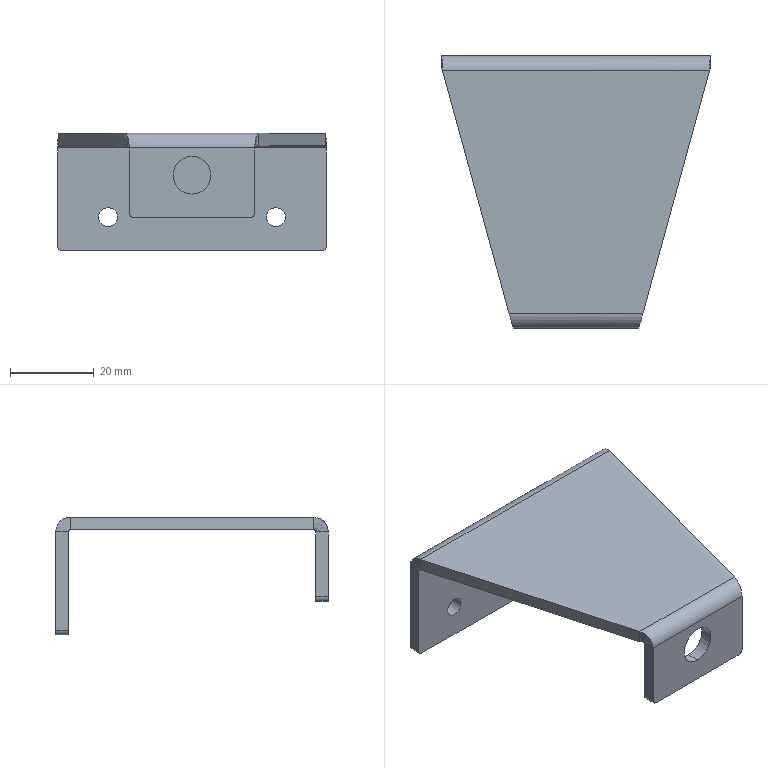Component | SolidWorks | SmallRoundCylinderBracket-1 | 1 solid | 32 faces | box 64 x 65 x 28 mm | volume 15113 mm3 | cylinder 14 | plane 14 | spline 4 | commonest cylinder face diameters 4.5 x4 2 x4 9 x2 7 x2 1 x2
STEP:
#1=CARTESIAN_POINT('',(2.534,-4.57,6.749));
#2=VERTEX_POINT('',#1);
#3=CARTESIAN_POINT('',(2.534,-4.57,6.395));
#4=VERTEX_POINT('',#3);
#5=CARTESIAN_POINT('',(2.534,-4.57,6.572));
#6=DIRECTION('',(0.,-1.,-0.));
#7=DIRECTION('',(0.,0.,-1.));
#8=AXIS2_PLACEMENT_3D('',#5,#6,#7);
#9=CIRCLE('',#8,0.1772);
#10=EDGE_CURVE('',#2,#4,#9,.T.);
#11=ORIENTED_EDGE('',*,*,#10,.F.);
#12=CARTESIAN_POINT('',(2.534,-4.688,6.749));
#13=VERTEX_POINT('',#12);
#14=CARTESIAN_POINT('',(2.534,-4.294,6.749));
#15=DIRECTION('',(0.,-1.,-0.));
#16=VECTOR('',#15,39.37);
#17=LINE('',#14,#16);
#18=EDGE_CURVE('',#2,#13,#17,.T.);
#19=ORIENTED_EDGE('',*,*,#18,.T.);
#20=CARTESIAN_POINT('',(2.534,-4.688,6.395));
#21=VERTEX_POINT('',#20);
#22=CARTESIAN_POINT('',(2.534,-4.688,6.572));
#23=DIRECTION('',(0.,-1.,-0.));
#24=DIRECTION('',(0.,0.,-1.));
#25=AXIS2_PLACEMENT_3D('',#22,#23,#24);
#26=CIRCLE('',#25,0.1772);
#27=EDGE_CURVE('',#13,#21,#26,.T.);
#28=ORIENTED_EDGE('',*,*,#27,.T.);
#29=CARTESIAN_POINT('',(2.534,-4.294,6.395));
#30=DIRECTION('',(0.,-1.,-0.));
#31=VECTOR('',#30,39.37);
#32=LINE('',#29,#31);
#33=EDGE_CURVE('',#4,#21,#32,.T.);
#34=ORIENTED_EDGE('',*,*,#33,.F.);
#35=EDGE_LOOP('',(#11,#19,#28,#34));
#36=FACE_OUTER_BOUND('',#35,.T.);
#37=CARTESIAN_POINT('',(2.534,-4.294,6.572));
#38=DIRECTION('',(0.,-1.,-0.));
#39=DIRECTION('',(0.,0.,-1.));
#40=AXIS2_PLACEMENT_3D('',#37,#38,#39);
#41=CYLINDRICAL_SURFACE('',#40,0.1772);
#42=ADVANCED_FACE('',(#36),#41,.F.);
#43=CARTESIAN_POINT('',(1.658,-2.247,6.178));
#44=VERTEX_POINT('',#43);
#45=CARTESIAN_POINT('',(1.835,-2.247,6.178));
#46=VERTEX_POINT('',#45);
#47=CARTESIAN_POINT('',(1.746,-2.247,6.178));
#48=DIRECTION('',(0.,1.,0.));
#49=DIRECTION('',(1.,0.,0.));
#50=AXIS2_PLACEMENT_3D('',#47,#48,#49);
#51=CIRCLE('',#50,0.08858);
#52=EDGE_CURVE('',#44,#46,#51,.T.);
#53=ORIENTED_EDGE('',*,*,#52,.F.);
#54=CARTESIAN_POINT('',(1.658,-2.129,6.178));
#55=VERTEX_POINT('',#54);
#56=CARTESIAN_POINT('',(1.658,-2.522,6.178));
#57=DIRECTION('',(0.,1.,0.));
#58=VECTOR('',#57,39.37);
#59=LINE('',#56,#58);
#60=EDGE_CURVE('',#44,#55,#59,.T.);
#61=ORIENTED_EDGE('',*,*,#60,.T.);
#62=CARTESIAN_POINT('',(1.835,-2.129,6.178));
#63=VERTEX_POINT('',#62);
#64=CARTESIAN_POINT('',(1.746,-2.129,6.178));
#65=DIRECTION('',(0.,1.,0.));
#66=DIRECTION('',(1.,0.,0.));
#67=AXIS2_PLACEMENT_3D('',#64,#65,#66);
#68=CIRCLE('',#67,0.08858);
#69=EDGE_CURVE('',#55,#63,#68,.T.);
#70=ORIENTED_EDGE('',*,*,#69,.T.);
#71=CARTESIAN_POINT('',(1.835,-2.522,6.178));
#72=DIRECTION('',(0.,1.,0.));
#73=VECTOR('',#72,39.37);
#74=LINE('',#71,#73);
#75=EDGE_CURVE('',#46,#63,#74,.T.);
#76=ORIENTED_EDGE('',*,*,#75,.F.);
#77=EDGE_LOOP('',(#53,#61,#70,#76));
#78=FACE_OUTER_BOUND('',#77,.T.);
#79=CARTESIAN_POINT('',(1.746,-2.522,6.178));
#80=DIRECTION('',(0.,1.,0.));
#81=DIRECTION('',(1.,0.,0.));
#82=AXIS2_PLACEMENT_3D('',#79,#80,#81);
#83=CYLINDRICAL_SURFACE('',#82,0.08858);
#84=ADVANCED_FACE('',(#78),#83,.F.);
#85=CARTESIAN_POINT('',(3.232,-2.247,6.178));
#86=VERTEX_POINT('',#85);
#87=CARTESIAN_POINT('',(3.41,-2.247,6.178));
#88=VERTEX_POINT('',#87);
#89=CARTESIAN_POINT('',(3.321,-2.247,6.178));
#90=DIRECTION('',(0.,1.,0.));
#91=DIRECTION('',(1.,0.,0.));
#92=AXIS2_PLACEMENT_3D('',#89,#90,#91);
#93=CIRCLE('',#92,0.08858);
#94=EDGE_CURVE('',#86,#88,#93,.T.);
#95=ORIENTED_EDGE('',*,*,#94,.F.);
#96=CARTESIAN_POINT('',(3.232,-2.129,6.178));
#97=VERTEX_POINT('',#96);
#98=CARTESIAN_POINT('',(3.232,-2.522,6.178));
#99=DIRECTION('',(0.,1.,0.));
#100=VECTOR('',#99,39.37);
#101=LINE('',#98,#100);
#102=EDGE_CURVE('',#86,#97,#101,.T.);
#103=ORIENTED_EDGE('',*,*,#102,.T.);
#104=CARTESIAN_POINT('',(3.41,-2.129,6.178));
#105=VERTEX_POINT('',#104);
#106=CARTESIAN_POINT('',(3.321,-2.129,6.178));
#107=DIRECTION('',(0.,1.,0.));
#108=DIRECTION('',(1.,0.,0.));
#109=AXIS2_PLACEMENT_3D('',#106,#107,#108);
#110=CIRCLE('',#109,0.08858);
#111=EDGE_CURVE('',#97,#105,#110,.T.);
#112=ORIENTED_EDGE('',*,*,#111,.T.);
#113=CARTESIAN_POINT('',(3.41,-2.522,6.178));
#114=DIRECTION('',(0.,1.,0.));
#115=VECTOR('',#114,39.37);
#116=LINE('',#113,#115);
#117=EDGE_CURVE('',#88,#105,#116,.T.);
#118=ORIENTED_EDGE('',*,*,#117,.F.);
#119=EDGE_LOOP('',(#95,#103,#112,#118));
#120=FACE_OUTER_BOUND('',#119,.T.);
#121=CARTESIAN_POINT('',(3.321,-2.522,6.178));
#122=DIRECTION('',(0.,1.,0.));
#123=DIRECTION('',(1.,0.,0.));
#124=AXIS2_PLACEMENT_3D('',#121,#122,#123);
#125=CYLINDRICAL_SURFACE('',#124,0.08858);
#126=ADVANCED_FACE('',(#120),#125,.F.);
#127=CARTESIAN_POINT('',(3.793,-2.129,6.828));
#128=VERTEX_POINT('',#127);
#129=CARTESIAN_POINT('',(1.274,-2.129,6.828));
#130=VERTEX_POINT('',#129);
#131=CARTESIAN_POINT('',(3.793,-2.129,6.828));
#132=DIRECTION('',(-1.,0.,0.));
#133=VECTOR('',#132,39.37);
#134=LINE('',#131,#133);
#135=EDGE_CURVE('',#128,#130,#134,.T.);
#136=ORIENTED_EDGE('',*,*,#135,.T.);
#137=CARTESIAN_POINT('',(1.279,-2.266,6.966));
#138=VERTEX_POINT('',#137);
#139=CARTESIAN_POINT('',(1.279,-2.266,6.966));
#140=CARTESIAN_POINT('',(1.276,-2.186,6.966));
#141=CARTESIAN_POINT('',(1.274,-2.129,6.909));
#142=CARTESIAN_POINT('',(1.274,-2.129,6.828));
#143=(BOUNDED_CURVE()B_SPLINE_CURVE(3,(#139,#140,#141,#142),.UNSPECIFIED.,.F.,.F.)B_SPLINE_CURVE_WITH_KNOTS((4,4),(4.712,6.283),.UNSPECIFIED.)CURVE()GEOMETRIC_REPRESENTATION_ITEM()RATIONAL_B_SPLINE_CURVE((1.,0.8047,0.8047,1.))REPRESENTATION_ITEM(''));
#144=EDGE_CURVE('',#138,#130,#143,.T.);
#145=ORIENTED_EDGE('',*,*,#144,.F.);
#146=CARTESIAN_POINT('',(3.788,-2.266,6.966));
#147=VERTEX_POINT('',#146);
#148=CARTESIAN_POINT('',(3.793,-2.266,6.966));
#149=DIRECTION('',(-1.,0.,0.));
#150=VECTOR('',#149,39.37);
#151=LINE('',#148,#150);
#152=EDGE_CURVE('',#147,#138,#151,.T.);
#153=ORIENTED_EDGE('',*,*,#152,.F.);
#154=CARTESIAN_POINT('',(3.793,-2.129,6.828));
#155=CARTESIAN_POINT('',(3.793,-2.129,6.909));
#156=CARTESIAN_POINT('',(3.791,-2.186,6.966));
#157=CARTESIAN_POINT('',(3.788,-2.266,6.966));
#158=(BOUNDED_CURVE()B_SPLINE_CURVE(3,(#154,#155,#156,#157),.UNSPECIFIED.,.F.,.F.)B_SPLINE_CURVE_WITH_KNOTS((4,4),(3.142,4.712),.UNSPECIFIED.)CURVE()GEOMETRIC_REPRESENTATION_ITEM()RATIONAL_B_SPLINE_CURVE((1.,0.8047,0.8047,1.))REPRESENTATION_ITEM(''));
#159=EDGE_CURVE('',#128,#147,#158,.T.);
#160=ORIENTED_EDGE('',*,*,#159,.F.);
#161=EDGE_LOOP('',(#136,#145,#153,#160));
#162=FACE_OUTER_BOUND('',#161,.T.);
#163=CARTESIAN_POINT('',(3.793,-2.266,6.828));
#164=DIRECTION('',(-1.,0.,0.));
#165=DIRECTION('',(0.,0.,1.));
#166=AXIS2_PLACEMENT_3D('',#163,#164,#165);
#167=CYLINDRICAL_SURFACE('',#166,0.1378);
#168=ADVANCED_FACE('',(#162),#167,.T.);
#169=ORIENTED_EDGE('',*,*,#152,.T.);
#170=CARTESIAN_POINT('',(1.905,-4.55,6.966));
#171=VERTEX_POINT('',#170);
#172=CARTESIAN_POINT('',(2.072,-5.16,6.966));
#173=DIRECTION('',(-0.2644,0.9644,0.));
#174=VECTOR('',#173,39.37);
#175=LINE('',#172,#174);
#176=EDGE_CURVE('',#171,#138,#175,.T.);
#177=ORIENTED_EDGE('',*,*,#176,.F.);
#178=CARTESIAN_POINT('',(3.162,-4.55,6.966));
#179=VERTEX_POINT('',#178);
#180=CARTESIAN_POINT('',(3.793,-4.55,6.966));
#181=DIRECTION('',(-1.,0.,0.));
#182=VECTOR('',#181,39.37);
#183=LINE('',#180,#182);
#184=EDGE_CURVE('',#179,#171,#183,.T.);
#185=ORIENTED_EDGE('',*,*,#184,.F.);
#186=CARTESIAN_POINT('',(3.171,-4.517,6.966));
#187=DIRECTION('',(-0.2644,-0.9644,0.));
#188=VECTOR('',#187,39.37);
#189=LINE('',#186,#188);
#190=EDGE_CURVE('',#147,#179,#189,.T.);
#191=ORIENTED_EDGE('',*,*,#190,.F.);
#192=EDGE_LOOP('',(#169,#177,#185,#191));
#193=FACE_OUTER_BOUND('',#192,.T.);
#194=CARTESIAN_POINT('',(3.793,-4.688,6.966));
#195=DIRECTION('',(0.,0.,1.));
#196=DIRECTION('',(1.,0.,0.));
#197=AXIS2_PLACEMENT_3D('',#194,#195,#196);
#198=PLANE('',#197);
#199=ADVANCED_FACE('',(#193),#198,.T.);
#200=ORIENTED_EDGE('',*,*,#184,.T.);
#201=CARTESIAN_POINT('',(1.943,-4.688,6.828));
#202=VERTEX_POINT('',#201);
#203=CARTESIAN_POINT('',(1.943,-4.688,6.828));
#204=CARTESIAN_POINT('',(1.943,-4.688,6.909));
#205=CARTESIAN_POINT('',(1.927,-4.631,6.966));
#206=CARTESIAN_POINT('',(1.905,-4.55,6.966));
#207=(BOUNDED_CURVE()B_SPLINE_CURVE(3,(#203,#204,#205,#206),.UNSPECIFIED.,.F.,.F.)B_SPLINE_CURVE_WITH_KNOTS((4,4),(3.142,4.712),.UNSPECIFIED.)CURVE()GEOMETRIC_REPRESENTATION_ITEM()RATIONAL_B_SPLINE_CURVE((1.,0.8047,0.8047,1.))REPRESENTATION_ITEM(''));
#208=EDGE_CURVE('',#202,#171,#207,.T.);
#209=ORIENTED_EDGE('',*,*,#208,.F.);
#210=CARTESIAN_POINT('',(3.124,-4.688,6.828));
#211=VERTEX_POINT('',#210);
#212=CARTESIAN_POINT('',(3.793,-4.688,6.828));
#213=DIRECTION('',(-1.,0.,0.));
#214=VECTOR('',#213,39.37);
#215=LINE('',#212,#214);
#216=EDGE_CURVE('',#211,#202,#215,.T.);
#217=ORIENTED_EDGE('',*,*,#216,.F.);
#218=CARTESIAN_POINT('',(3.162,-4.55,6.966));
#219=CARTESIAN_POINT('',(3.14,-4.631,6.966));
#220=CARTESIAN_POINT('',(3.124,-4.688,6.909));
#221=CARTESIAN_POINT('',(3.124,-4.688,6.828));
#222=(BOUNDED_CURVE()B_SPLINE_CURVE(3,(#218,#219,#220,#221),.UNSPECIFIED.,.F.,.F.)B_SPLINE_CURVE_WITH_KNOTS((4,4),(4.712,6.283),.UNSPECIFIED.)CURVE()GEOMETRIC_REPRESENTATION_ITEM()RATIONAL_B_SPLINE_CURVE((1.,0.8047,0.8047,1.))REPRESENTATION_ITEM(''));
#223=EDGE_CURVE('',#179,#211,#222,.T.);
#224=ORIENTED_EDGE('',*,*,#223,.F.);
#225=EDGE_LOOP('',(#200,#209,#217,#224));
#226=FACE_OUTER_BOUND('',#225,.T.);
#227=CARTESIAN_POINT('',(3.793,-4.55,6.828));
#228=DIRECTION('',(-1.,0.,0.));
#229=DIRECTION('',(0.,0.,1.));
#230=AXIS2_PLACEMENT_3D('',#227,#228,#229);
#231=CYLINDRICAL_SURFACE('',#230,0.1378);
#232=ADVANCED_FACE('',(#226),#231,.T.);
#233=CARTESIAN_POINT('',(2.534,-4.688,6.572));
#234=DIRECTION('',(0.,-1.,-0.));
#235=DIRECTION('',(0.,0.,-1.));
#236=AXIS2_PLACEMENT_3D('',#233,#234,#235);
#237=CIRCLE('',#236,0.1772);
#238=EDGE_CURVE('',#21,#13,#237,.T.);
#239=ORIENTED_EDGE('',*,*,#238,.F.);
#240=ORIENTED_EDGE('',*,*,#27,.F.);
#241=EDGE_LOOP('',(#239,#240));
#242=FACE_BOUND('',#241,.T.);
#243=CARTESIAN_POINT('',(1.943,-4.688,6.218));
#244=VERTEX_POINT('',#243);
#245=CARTESIAN_POINT('',(1.943,-4.688,8.226));
#246=DIRECTION('',(0.,0.,-1.));
#247=VECTOR('',#246,39.37);
#248=LINE('',#245,#247);
#249=EDGE_CURVE('',#202,#244,#248,.T.);
#250=ORIENTED_EDGE('',*,*,#249,.T.);
#251=CARTESIAN_POINT('',(1.982,-4.688,6.178));
#252=VERTEX_POINT('',#251);
#253=CARTESIAN_POINT('',(1.982,-4.688,6.218));
#254=DIRECTION('',(0.,-1.,-0.));
#255=DIRECTION('',(0.,0.,-1.));
#256=AXIS2_PLACEMENT_3D('',#253,#254,#255);
#257=CIRCLE('',#256,0.03937);
#258=EDGE_CURVE('',#244,#252,#257,.T.);
#259=ORIENTED_EDGE('',*,*,#258,.T.);
#260=CARTESIAN_POINT('',(3.085,-4.688,6.178));
#261=VERTEX_POINT('',#260);
#262=CARTESIAN_POINT('',(3.793,-4.688,6.178));
#263=DIRECTION('',(-1.,0.,0.));
#264=VECTOR('',#263,39.37);
#265=LINE('',#262,#264);
#266=EDGE_CURVE('',#261,#252,#265,.T.);
#267=ORIENTED_EDGE('',*,*,#266,.F.);
#268=CARTESIAN_POINT('',(3.124,-4.688,6.218));
#269=VERTEX_POINT('',#268);
#270=CARTESIAN_POINT('',(3.085,-4.688,6.218));
#271=DIRECTION('',(0.,-1.,-0.));
#272=DIRECTION('',(0.,0.,-1.));
#273=AXIS2_PLACEMENT_3D('',#270,#271,#272);
#274=CIRCLE('',#273,0.03937);
#275=EDGE_CURVE('',#261,#269,#274,.T.);
#276=ORIENTED_EDGE('',*,*,#275,.T.);
#277=CARTESIAN_POINT('',(3.124,-4.688,8.226));
#278=DIRECTION('',(0.,0.,-1.));
#279=VECTOR('',#278,39.37);
#280=LINE('',#277,#279);
#281=EDGE_CURVE('',#211,#269,#280,.T.);
#282=ORIENTED_EDGE('',*,*,#281,.F.);
#283=ORIENTED_EDGE('',*,*,#216,.T.);
#284=EDGE_LOOP('',(#250,#259,#267,#276,#282,#283));
#285=FACE_OUTER_BOUND('',#284,.T.);
#286=CARTESIAN_POINT('',(3.793,-4.688,6.178));
#287=DIRECTION('',(0.,-1.,-0.));
#288=DIRECTION('',(0.,0.,-1.));
#289=AXIS2_PLACEMENT_3D('',#286,#287,#288);
#290=PLANE('',#289);
#291=ADVANCED_FACE('',(#242,#285),#290,.T.);
#292=ORIENTED_EDGE('',*,*,#266,.T.);
#293=CARTESIAN_POINT('',(1.982,-4.57,6.178));
#294=VERTEX_POINT('',#293);
#295=CARTESIAN_POINT('',(1.982,-4.57,6.178));
#296=DIRECTION('',(0.,1.,0.));
#297=VECTOR('',#296,39.37);
#298=LINE('',#295,#297);
#299=EDGE_CURVE('',#252,#294,#298,.T.);
#300=ORIENTED_EDGE('',*,*,#299,.T.);
#301=CARTESIAN_POINT('',(3.085,-4.57,6.178));
#302=VERTEX_POINT('',#301);
#303=CARTESIAN_POINT('',(3.793,-4.57,6.178));
#304=DIRECTION('',(-1.,0.,0.));
#305=VECTOR('',#304,39.37);
#306=LINE('',#303,#305);
#307=EDGE_CURVE('',#302,#294,#306,.T.);
#308=ORIENTED_EDGE('',*,*,#307,.F.);
#309=CARTESIAN_POINT('',(3.085,-4.57,6.178));
#310=DIRECTION('',(0.,-1.,-0.));
#311=VECTOR('',#310,39.37);
#312=LINE('',#309,#311);
#313=EDGE_CURVE('',#302,#261,#312,.T.);
#314=ORIENTED_EDGE('',*,*,#313,.T.);
#315=EDGE_LOOP('',(#292,#300,#308,#314));
#316=FACE_OUTER_BOUND('',#315,.T.);
#317=CARTESIAN_POINT('',(3.793,-4.57,6.178));
#318=DIRECTION('',(0.,0.,-1.));
#319=DIRECTION('',(0.,1.,0.));
#320=AXIS2_PLACEMENT_3D('',#317,#318,#319);
#321=PLANE('',#320);
#322=ADVANCED_FACE('',(#316),#321,.T.);
#323=CARTESIAN_POINT('',(2.534,-4.57,6.572));
#324=DIRECTION('',(0.,-1.,-0.));
#325=DIRECTION('',(0.,0.,-1.));
#326=AXIS2_PLACEMENT_3D('',#323,#324,#325);
#327=CIRCLE('',#326,0.1772);
#328=EDGE_CURVE('',#4,#2,#327,.T.);
#329=ORIENTED_EDGE('',*,*,#328,.T.);
#330=ORIENTED_EDGE('',*,*,#10,.T.);
#331=EDGE_LOOP('',(#329,#330));
#332=FACE_BOUND('',#331,.T.);
#333=ORIENTED_EDGE('',*,*,#307,.T.);
#334=CARTESIAN_POINT('',(1.943,-4.57,6.218));
#335=VERTEX_POINT('',#334);
#336=CARTESIAN_POINT('',(1.982,-4.57,6.218));
#337=DIRECTION('',(0.,1.,0.));
#338=DIRECTION('',(0.,0.,-1.));
#339=AXIS2_PLACEMENT_3D('',#336,#337,#338);
#340=CIRCLE('',#339,0.03937);
#341=EDGE_CURVE('',#294,#335,#340,.T.);
#342=ORIENTED_EDGE('',*,*,#341,.T.);
#343=CARTESIAN_POINT('',(1.943,-4.57,6.828));
#344=VERTEX_POINT('',#343);
#345=CARTESIAN_POINT('',(1.943,-4.57,6.178));
#346=DIRECTION('',(0.,0.,-1.));
#347=VECTOR('',#346,39.37);
#348=LINE('',#345,#347);
#349=EDGE_CURVE('',#344,#335,#348,.T.);
#350=ORIENTED_EDGE('',*,*,#349,.F.);
#351=CARTESIAN_POINT('',(3.124,-4.57,6.828));
#352=VERTEX_POINT('',#351);
#353=CARTESIAN_POINT('',(3.793,-4.57,6.828));
#354=DIRECTION('',(-1.,0.,0.));
#355=VECTOR('',#354,39.37);
#356=LINE('',#353,#355);
#357=EDGE_CURVE('',#352,#344,#356,.T.);
#358=ORIENTED_EDGE('',*,*,#357,.F.);
#359=CARTESIAN_POINT('',(3.124,-4.57,6.218));
#360=VERTEX_POINT('',#359);
#361=CARTESIAN_POINT('',(3.124,-4.57,6.178));
#362=DIRECTION('',(0.,0.,-1.));
#363=VECTOR('',#362,39.37);
#364=LINE('',#361,#363);
#365=EDGE_CURVE('',#352,#360,#364,.T.);
#366=ORIENTED_EDGE('',*,*,#365,.T.);
#367=CARTESIAN_POINT('',(3.085,-4.57,6.218));
#368=DIRECTION('',(0.,1.,0.));
#369=DIRECTION('',(0.,0.,-1.));
#370=AXIS2_PLACEMENT_3D('',#367,#368,#369);
#371=CIRCLE('',#370,0.03937);
#372=EDGE_CURVE('',#360,#302,#371,.T.);
#373=ORIENTED_EDGE('',*,*,#372,.T.);
#374=EDGE_LOOP('',(#333,#342,#350,#358,#366,#373));
#375=FACE_OUTER_BOUND('',#374,.T.);
#376=CARTESIAN_POINT('',(3.793,-4.57,6.178));
#377=DIRECTION('',(0.,-1.,-0.));
#378=DIRECTION('',(0.,0.,-1.));
#379=AXIS2_PLACEMENT_3D('',#376,#377,#378);
#380=PLANE('',#379);
#381=ADVANCED_FACE('',(#332,#375),#380,.F.);
#382=CARTESIAN_POINT('',(1.905,-4.55,6.848));
#383=VERTEX_POINT('',#382);
#384=CARTESIAN_POINT('',(1.943,-4.57,6.828));
#385=CARTESIAN_POINT('',(1.943,-4.57,6.84));
#386=CARTESIAN_POINT('',(1.927,-4.561,6.848));
#387=CARTESIAN_POINT('',(1.905,-4.55,6.848));
#388=(BOUNDED_CURVE()B_SPLINE_CURVE(3,(#384,#385,#386,#387),.UNSPECIFIED.,.F.,.F.)B_SPLINE_CURVE_WITH_KNOTS((4,4),(3.142,4.712),.UNSPECIFIED.)CURVE()GEOMETRIC_REPRESENTATION_ITEM()RATIONAL_B_SPLINE_CURVE((1.,0.8047,0.8047,1.))REPRESENTATION_ITEM(''));
#389=EDGE_CURVE('',#344,#383,#388,.T.);
#390=ORIENTED_EDGE('',*,*,#389,.T.);
#391=CARTESIAN_POINT('',(3.162,-4.55,6.848));
#392=VERTEX_POINT('',#391);
#393=CARTESIAN_POINT('',(3.793,-4.55,6.848));
#394=DIRECTION('',(-1.,0.,0.));
#395=VECTOR('',#394,39.37);
#396=LINE('',#393,#395);
#397=EDGE_CURVE('',#392,#383,#396,.T.);
#398=ORIENTED_EDGE('',*,*,#397,.F.);
#399=CARTESIAN_POINT('',(3.162,-4.55,6.848));
#400=CARTESIAN_POINT('',(3.14,-4.561,6.848));
#401=CARTESIAN_POINT('',(3.124,-4.57,6.84));
#402=CARTESIAN_POINT('',(3.124,-4.57,6.828));
#403=(BOUNDED_CURVE()B_SPLINE_CURVE(3,(#399,#400,#401,#402),.UNSPECIFIED.,.F.,.F.)B_SPLINE_CURVE_WITH_KNOTS((4,4),(4.712,6.283),.UNSPECIFIED.)CURVE()GEOMETRIC_REPRESENTATION_ITEM()RATIONAL_B_SPLINE_CURVE((1.,0.8047,0.8047,1.))REPRESENTATION_ITEM(''));
#404=EDGE_CURVE('',#392,#352,#403,.T.);
#405=ORIENTED_EDGE('',*,*,#404,.T.);
#406=ORIENTED_EDGE('',*,*,#357,.T.);
#407=EDGE_LOOP('',(#390,#398,#405,#406));
#408=FACE_OUTER_BOUND('',#407,.T.);
#409=CARTESIAN_POINT('',(3.793,-4.55,6.828));
#410=DIRECTION('',(-1.,0.,0.));
#411=DIRECTION('',(0.,0.,1.));
#412=AXIS2_PLACEMENT_3D('',#409,#410,#411);
#413=CYLINDRICAL_SURFACE('',#412,0.01969);
#414=ADVANCED_FACE('',(#408),#413,.F.);
#415=CARTESIAN_POINT('',(1.279,-2.266,6.848));
#416=VERTEX_POINT('',#415);
#417=CARTESIAN_POINT('',(2.072,-5.16,6.848));
#418=DIRECTION('',(-0.2644,0.9644,0.));
#419=VECTOR('',#418,39.37);
#420=LINE('',#417,#419);
#421=EDGE_CURVE('',#383,#416,#420,.T.);
#422=ORIENTED_EDGE('',*,*,#421,.T.);
#423=CARTESIAN_POINT('',(3.788,-2.266,6.848));
#424=VERTEX_POINT('',#423);
#425=CARTESIAN_POINT('',(3.793,-2.266,6.848));
#426=DIRECTION('',(-1.,0.,0.));
#427=VECTOR('',#426,39.37);
#428=LINE('',#425,#427);
#429=EDGE_CURVE('',#424,#416,#428,.T.);
#430=ORIENTED_EDGE('',*,*,#429,.F.);
#431=CARTESIAN_POINT('',(3.171,-4.517,6.848));
#432=DIRECTION('',(-0.2644,-0.9644,0.));
#433=VECTOR('',#432,39.37);
#434=LINE('',#431,#433);
#435=EDGE_CURVE('',#424,#392,#434,.T.);
#436=ORIENTED_EDGE('',*,*,#435,.T.);
#437=ORIENTED_EDGE('',*,*,#397,.T.);
#438=EDGE_LOOP('',(#422,#430,#436,#437));
#439=FACE_OUTER_BOUND('',#438,.T.);
#440=CARTESIAN_POINT('',(3.793,-4.688,6.848));
#441=DIRECTION('',(0.,0.,1.));
#442=DIRECTION('',(1.,0.,0.));
#443=AXIS2_PLACEMENT_3D('',#440,#441,#442);
#444=PLANE('',#443);
#445=ADVANCED_FACE('',(#439),#444,.F.);
#446=CARTESIAN_POINT('',(1.274,-2.247,6.828));
#447=VERTEX_POINT('',#446);
#448=CARTESIAN_POINT('',(1.279,-2.266,6.848));
#449=CARTESIAN_POINT('',(1.276,-2.255,6.848));
#450=CARTESIAN_POINT('',(1.274,-2.247,6.84));
#451=CARTESIAN_POINT('',(1.274,-2.247,6.828));
#452=(BOUNDED_CURVE()B_SPLINE_CURVE(3,(#448,#449,#450,#451),.UNSPECIFIED.,.F.,.F.)B_SPLINE_CURVE_WITH_KNOTS((4,4),(4.712,6.283),.UNSPECIFIED.)CURVE()GEOMETRIC_REPRESENTATION_ITEM()RATIONAL_B_SPLINE_CURVE((1.,0.8047,0.8047,1.))REPRESENTATION_ITEM(''));
#453=EDGE_CURVE('',#416,#447,#452,.T.);
#454=ORIENTED_EDGE('',*,*,#453,.T.);
#455=CARTESIAN_POINT('',(3.793,-2.247,6.828));
#456=VERTEX_POINT('',#455);
#457=CARTESIAN_POINT('',(3.793,-2.247,6.828));
#458=DIRECTION('',(-1.,0.,0.));
#459=VECTOR('',#458,39.37);
#460=LINE('',#457,#459);
#461=EDGE_CURVE('',#456,#447,#460,.T.);
#462=ORIENTED_EDGE('',*,*,#461,.F.);
#463=CARTESIAN_POINT('',(3.793,-2.247,6.828));
#464=CARTESIAN_POINT('',(3.793,-2.247,6.84));
#465=CARTESIAN_POINT('',(3.791,-2.255,6.848));
#466=CARTESIAN_POINT('',(3.788,-2.266,6.848));
#467=(BOUNDED_CURVE()B_SPLINE_CURVE(3,(#463,#464,#465,#466),.UNSPECIFIED.,.F.,.F.)B_SPLINE_CURVE_WITH_KNOTS((4,4),(3.142,4.712),.UNSPECIFIED.)CURVE()GEOMETRIC_REPRESENTATION_ITEM()RATIONAL_B_SPLINE_CURVE((1.,0.8047,0.8047,1.))REPRESENTATION_ITEM(''));
#468=EDGE_CURVE('',#456,#424,#467,.T.);
#469=ORIENTED_EDGE('',*,*,#468,.T.);
#470=ORIENTED_EDGE('',*,*,#429,.T.);
#471=EDGE_LOOP('',(#454,#462,#469,#470));
#472=FACE_OUTER_BOUND('',#471,.T.);
#473=CARTESIAN_POINT('',(3.793,-2.266,6.828));
#474=DIRECTION('',(-1.,0.,0.));
#475=DIRECTION('',(0.,0.,1.));
#476=AXIS2_PLACEMENT_3D('',#473,#474,#475);
#477=CYLINDRICAL_SURFACE('',#476,0.01969);
#478=ADVANCED_FACE('',(#472),#477,.F.);
#479=CARTESIAN_POINT('',(3.793,-2.247,5.903));
#480=VERTEX_POINT('',#479);
#481=CARTESIAN_POINT('',(3.793,-2.247,6.966));
#482=DIRECTION('',(0.,0.,-1.));
#483=VECTOR('',#482,39.37);
#484=LINE('',#481,#483);
#485=EDGE_CURVE('',#456,#480,#484,.T.);
#486=ORIENTED_EDGE('',*,*,#485,.T.);
#487=CARTESIAN_POINT('',(3.793,-2.129,5.903));
#488=VERTEX_POINT('',#487);
#489=CARTESIAN_POINT('',(3.793,-2.266,5.903));
#490=DIRECTION('',(0.,1.,0.));
#491=VECTOR('',#490,39.37);
#492=LINE('',#489,#491);
#493=EDGE_CURVE('',#480,#488,#492,.T.);
#494=ORIENTED_EDGE('',*,*,#493,.T.);
#495=CARTESIAN_POINT('',(3.793,-2.129,6.966));
#496=DIRECTION('',(0.,0.,-1.));
#497=VECTOR('',#496,39.37);
#498=LINE('',#495,#497);
#499=EDGE_CURVE('',#128,#488,#498,.T.);
#500=ORIENTED_EDGE('',*,*,#499,.F.);
#501=CARTESIAN_POINT('',(3.793,-2.129,6.828));
#502=DIRECTION('',(0.,-1.,0.));
#503=VECTOR('',#502,39.37);
#504=LINE('',#501,#503);
#505=EDGE_CURVE('',#128,#456,#504,.T.);
#506=ORIENTED_EDGE('',*,*,#505,.T.);
#507=EDGE_LOOP('',(#486,#494,#500,#506));
#508=FACE_OUTER_BOUND('',#507,.T.);
#509=CARTESIAN_POINT('',(3.793,-2.266,6.848));
#510=DIRECTION('',(1.,0.,0.));
#511=DIRECTION('',(0.,0.,-1.));
#512=AXIS2_PLACEMENT_3D('',#509,#510,#511);
#513=PLANE('',#512);
#514=ADVANCED_FACE('',(#508),#513,.T.);
#515=CARTESIAN_POINT('',(1.746,-2.247,6.178));
#516=DIRECTION('',(0.,1.,0.));
#517=DIRECTION('',(1.,0.,0.));
#518=AXIS2_PLACEMENT_3D('',#515,#516,#517);
#519=CIRCLE('',#518,0.08858);
#520=EDGE_CURVE('',#46,#44,#519,.T.);
#521=ORIENTED_EDGE('',*,*,#520,.T.);
#522=ORIENTED_EDGE('',*,*,#52,.T.);
#523=EDGE_LOOP('',(#521,#522));
#524=FACE_BOUND('',#523,.T.);
#525=CARTESIAN_POINT('',(3.321,-2.247,6.178));
#526=DIRECTION('',(0.,1.,0.));
#527=DIRECTION('',(1.,0.,0.));
#528=AXIS2_PLACEMENT_3D('',#525,#526,#527);
#529=CIRCLE('',#528,0.08858);
#530=EDGE_CURVE('',#88,#86,#529,.T.);
#531=ORIENTED_EDGE('',*,*,#530,.T.);
#532=ORIENTED_EDGE('',*,*,#94,.T.);
#533=EDGE_LOOP('',(#531,#532));
#534=FACE_BOUND('',#533,.T.);
#535=CARTESIAN_POINT('',(3.754,-2.247,5.863));
#536=VERTEX_POINT('',#535);
#537=CARTESIAN_POINT('',(1.313,-2.247,5.863));
#538=VERTEX_POINT('',#537);
#539=CARTESIAN_POINT('',(3.793,-2.247,5.863));
#540=DIRECTION('',(-1.,0.,0.));
#541=VECTOR('',#540,39.37);
#542=LINE('',#539,#541);
#543=EDGE_CURVE('',#536,#538,#542,.T.);
#544=ORIENTED_EDGE('',*,*,#543,.F.);
#545=CARTESIAN_POINT('',(3.754,-2.247,5.903));
#546=DIRECTION('',(0.,-1.,0.));
#547=DIRECTION('',(1.,0.,0.));
#548=AXIS2_PLACEMENT_3D('',#545,#546,#547);
#549=CIRCLE('',#548,0.03937);
#550=EDGE_CURVE('',#536,#480,#549,.T.);
#551=ORIENTED_EDGE('',*,*,#550,.T.);
#552=ORIENTED_EDGE('',*,*,#485,.F.);
#553=ORIENTED_EDGE('',*,*,#461,.T.);
#554=CARTESIAN_POINT('',(1.274,-2.247,5.903));
#555=VERTEX_POINT('',#554);
#556=CARTESIAN_POINT('',(1.274,-2.247,6.966));
#557=DIRECTION('',(0.,0.,-1.));
#558=VECTOR('',#557,39.37);
#559=LINE('',#556,#558);
#560=EDGE_CURVE('',#447,#555,#559,.T.);
#561=ORIENTED_EDGE('',*,*,#560,.T.);
#562=CARTESIAN_POINT('',(1.313,-2.247,5.903));
#563=DIRECTION('',(0.,-1.,0.));
#564=DIRECTION('',(1.,0.,0.));
#565=AXIS2_PLACEMENT_3D('',#562,#563,#564);
#566=CIRCLE('',#565,0.03937);
#567=EDGE_CURVE('',#555,#538,#566,.T.);
#568=ORIENTED_EDGE('',*,*,#567,.T.);
#569=EDGE_LOOP('',(#544,#551,#552,#553,#561,#568));
#570=FACE_OUTER_BOUND('',#569,.T.);
#571=CARTESIAN_POINT('',(3.793,-2.247,6.966));
#572=DIRECTION('',(0.,1.,0.));
#573=DIRECTION('',(1.,0.,0.));
#574=AXIS2_PLACEMENT_3D('',#571,#572,#573);
#575=PLANE('',#574);
#576=ADVANCED_FACE('',(#524,#534,#570),#575,.F.);
#577=CARTESIAN_POINT('',(3.754,-2.129,5.863));
#578=VERTEX_POINT('',#577);
#579=CARTESIAN_POINT('',(1.313,-2.129,5.863));
#580=VERTEX_POINT('',#579);
#581=CARTESIAN_POINT('',(3.793,-2.129,5.863));
#582=DIRECTION('',(-1.,0.,0.));
#583=VECTOR('',#582,39.37);
#584=LINE('',#581,#583);
#585=EDGE_CURVE('',#578,#580,#584,.T.);
#586=ORIENTED_EDGE('',*,*,#585,.F.);
#587=CARTESIAN_POINT('',(3.754,-2.129,5.863));
#588=DIRECTION('',(0.,-1.,0.));
#589=VECTOR('',#588,39.37);
#590=LINE('',#587,#589);
#591=EDGE_CURVE('',#578,#536,#590,.T.);
#592=ORIENTED_EDGE('',*,*,#591,.T.);
#593=ORIENTED_EDGE('',*,*,#543,.T.);
#594=CARTESIAN_POINT('',(1.313,-2.129,5.863));
#595=DIRECTION('',(0.,1.,0.));
#596=VECTOR('',#595,39.37);
#597=LINE('',#594,#596);
#598=EDGE_CURVE('',#538,#580,#597,.T.);
#599=ORIENTED_EDGE('',*,*,#598,.T.);
#600=EDGE_LOOP('',(#586,#592,#593,#599));
#601=FACE_OUTER_BOUND('',#600,.T.);
#602=CARTESIAN_POINT('',(3.793,-2.129,5.863));
#603=DIRECTION('',(0.,0.,-1.));
#604=DIRECTION('',(-1.,0.,0.));
#605=AXIS2_PLACEMENT_3D('',#602,#603,#604);
#606=PLANE('',#605);
#607=ADVANCED_FACE('',(#601),#606,.T.);
#608=CARTESIAN_POINT('',(1.746,-2.129,6.178));
#609=DIRECTION('',(0.,1.,0.));
#610=DIRECTION('',(1.,0.,0.));
#611=AXIS2_PLACEMENT_3D('',#608,#609,#610);
#612=CIRCLE('',#611,0.08858);
#613=EDGE_CURVE('',#63,#55,#612,.T.);
#614=ORIENTED_EDGE('',*,*,#613,.F.);
#615=ORIENTED_EDGE('',*,*,#69,.F.);
#616=EDGE_LOOP('',(#614,#615));
#617=FACE_BOUND('',#616,.T.);
#618=CARTESIAN_POINT('',(3.321,-2.129,6.178));
#619=DIRECTION('',(0.,1.,0.));
#620=DIRECTION('',(1.,0.,0.));
#621=AXIS2_PLACEMENT_3D('',#618,#619,#620);
#622=CIRCLE('',#621,0.08858);
#623=EDGE_CURVE('',#105,#97,#622,.T.);
#624=ORIENTED_EDGE('',*,*,#623,.F.);
#625=ORIENTED_EDGE('',*,*,#111,.F.);
#626=EDGE_LOOP('',(#624,#625));
#627=FACE_BOUND('',#626,.T.);
#628=ORIENTED_EDGE('',*,*,#499,.T.);
#629=CARTESIAN_POINT('',(3.754,-2.129,5.903));
#630=DIRECTION('',(0.,1.,0.));
#631=DIRECTION('',(1.,0.,0.));
#632=AXIS2_PLACEMENT_3D('',#629,#630,#631);
#633=CIRCLE('',#632,0.03937);
#634=EDGE_CURVE('',#488,#578,#633,.T.);
#635=ORIENTED_EDGE('',*,*,#634,.T.);
#636=ORIENTED_EDGE('',*,*,#585,.T.);
#637=CARTESIAN_POINT('',(1.274,-2.129,5.903));
#638=VERTEX_POINT('',#637);
#639=CARTESIAN_POINT('',(1.313,-2.129,5.903));
#640=DIRECTION('',(0.,1.,0.));
#641=DIRECTION('',(1.,0.,0.));
#642=AXIS2_PLACEMENT_3D('',#639,#640,#641);
#643=CIRCLE('',#642,0.03937);
#644=EDGE_CURVE('',#580,#638,#643,.T.);
#645=ORIENTED_EDGE('',*,*,#644,.T.);
#646=CARTESIAN_POINT('',(1.274,-2.129,6.966));
#647=DIRECTION('',(0.,0.,-1.));
#648=VECTOR('',#647,39.37);
#649=LINE('',#646,#648);
#650=EDGE_CURVE('',#130,#638,#649,.T.);
#651=ORIENTED_EDGE('',*,*,#650,.F.);
#652=ORIENTED_EDGE('',*,*,#135,.F.);
#653=EDGE_LOOP('',(#628,#635,#636,#645,#651,#652));
#654=FACE_OUTER_BOUND('',#653,.T.);
#655=CARTESIAN_POINT('',(3.793,-2.129,6.966));
#656=DIRECTION('',(0.,1.,0.));
#657=DIRECTION('',(1.,0.,0.));
#658=AXIS2_PLACEMENT_3D('',#655,#656,#657);
#659=PLANE('',#658);
#660=ADVANCED_FACE('',(#617,#627,#654),#659,.T.);
#661=ORIENTED_EDGE('',*,*,#650,.T.);
#662=CARTESIAN_POINT('',(1.274,-2.247,5.903));
#663=DIRECTION('',(0.,-1.,0.));
#664=VECTOR('',#663,39.37);
#665=LINE('',#662,#664);
#666=EDGE_CURVE('',#638,#555,#665,.T.);
#667=ORIENTED_EDGE('',*,*,#666,.T.);
#668=ORIENTED_EDGE('',*,*,#560,.F.);
#669=CARTESIAN_POINT('',(1.274,-2.247,6.828));
#670=DIRECTION('',(0.,1.,0.));
#671=VECTOR('',#670,39.37);
#672=LINE('',#669,#671);
#673=EDGE_CURVE('',#447,#130,#672,.T.);
#674=ORIENTED_EDGE('',*,*,#673,.T.);
#675=EDGE_LOOP('',(#661,#667,#668,#674));
#676=FACE_OUTER_BOUND('',#675,.T.);
#677=CARTESIAN_POINT('',(1.274,-2.266,6.828));
#678=DIRECTION('',(1.,0.,0.));
#679=DIRECTION('',(0.,0.,-1.));
#680=AXIS2_PLACEMENT_3D('',#677,#678,#679);
#681=PLANE('',#680);
#682=ADVANCED_FACE('',(#676),#681,.F.);
#683=CARTESIAN_POINT('',(3.162,-4.55,6.848));
#684=DIRECTION('',(0.,0.,1.));
#685=VECTOR('',#684,39.37);
#686=LINE('',#683,#685);
#687=EDGE_CURVE('',#392,#179,#686,.T.);
#688=ORIENTED_EDGE('',*,*,#687,.F.);
#689=ORIENTED_EDGE('',*,*,#435,.F.);
#690=CARTESIAN_POINT('',(3.788,-2.266,6.848));
#691=DIRECTION('',(0.,0.,1.));
#692=VECTOR('',#691,39.37);
#693=LINE('',#690,#692);
#694=EDGE_CURVE('',#424,#147,#693,.T.);
#695=ORIENTED_EDGE('',*,*,#694,.T.);
#696=ORIENTED_EDGE('',*,*,#190,.T.);
#697=EDGE_LOOP('',(#688,#689,#695,#696));
#698=FACE_OUTER_BOUND('',#697,.T.);
#699=CARTESIAN_POINT('',(3.171,-4.517,6.848));
#700=DIRECTION('',(-0.9644,0.2644,0.));
#701=DIRECTION('',(-0.2644,-0.9644,0.));
#702=AXIS2_PLACEMENT_3D('',#699,#700,#701);
#703=PLANE('',#702);
#704=ADVANCED_FACE('',(#698),#703,.F.);
#705=ORIENTED_EDGE('',*,*,#281,.T.);
#706=CARTESIAN_POINT('',(3.124,-4.688,6.218));
#707=DIRECTION('',(0.,1.,0.));
#708=VECTOR('',#707,39.37);
#709=LINE('',#706,#708);
#710=EDGE_CURVE('',#269,#360,#709,.T.);
#711=ORIENTED_EDGE('',*,*,#710,.T.);
#712=ORIENTED_EDGE('',*,*,#365,.F.);
#713=CARTESIAN_POINT('',(3.124,-4.688,6.828));
#714=DIRECTION('',(0.,1.,0.));
#715=VECTOR('',#714,39.37);
#716=LINE('',#713,#715);
#717=EDGE_CURVE('',#211,#352,#716,.T.);
#718=ORIENTED_EDGE('',*,*,#717,.F.);
#719=EDGE_LOOP('',(#705,#711,#712,#718));
#720=FACE_OUTER_BOUND('',#719,.T.);
#721=CARTESIAN_POINT('',(3.124,-4.688,8.226));
#722=DIRECTION('',(-1.,0.,0.));
#723=DIRECTION('',(0.,0.,-1.));
#724=AXIS2_PLACEMENT_3D('',#721,#722,#723);
#725=PLANE('',#724);
#726=ADVANCED_FACE('',(#720),#725,.F.);
#727=ORIENTED_EDGE('',*,*,#223,.T.);
#728=ORIENTED_EDGE('',*,*,#717,.T.);
#729=ORIENTED_EDGE('',*,*,#404,.F.);
#730=ORIENTED_EDGE('',*,*,#687,.T.);
#731=EDGE_LOOP('',(#727,#728,#729,#730));
#732=FACE_OUTER_BOUND('',#731,.T.);
#733=CARTESIAN_POINT('',(3.124,-4.688,6.828));
#734=CARTESIAN_POINT('',(3.124,-4.648,6.828));
#735=CARTESIAN_POINT('',(3.124,-4.609,6.828));
#736=CARTESIAN_POINT('',(3.124,-4.57,6.828));
#737=CARTESIAN_POINT('',(3.124,-4.688,6.552));
#738=CARTESIAN_POINT('',(3.124,-4.648,6.631));
#739=CARTESIAN_POINT('',(3.124,-4.609,6.71));
#740=CARTESIAN_POINT('',(3.124,-4.57,6.789));
#741=CARTESIAN_POINT('',(3.2,-4.412,6.552));
#742=CARTESIAN_POINT('',(3.2,-4.451,6.631));
#743=CARTESIAN_POINT('',(3.2,-4.491,6.71));
#744=CARTESIAN_POINT('',(3.2,-4.53,6.789));
#745=CARTESIAN_POINT('',(3.2,-4.412,6.828));
#746=CARTESIAN_POINT('',(3.2,-4.451,6.828));
#747=CARTESIAN_POINT('',(3.2,-4.491,6.828));
#748=CARTESIAN_POINT('',(3.2,-4.53,6.828));
#749=CARTESIAN_POINT('',(3.2,-4.412,7.104));
#750=CARTESIAN_POINT('',(3.2,-4.451,7.025));
#751=CARTESIAN_POINT('',(3.2,-4.491,6.946));
#752=CARTESIAN_POINT('',(3.2,-4.53,6.867));
#753=CARTESIAN_POINT('',(3.124,-4.688,7.104));
#754=CARTESIAN_POINT('',(3.124,-4.648,7.025));
#755=CARTESIAN_POINT('',(3.124,-4.609,6.946));
#756=CARTESIAN_POINT('',(3.124,-4.57,6.867));
#757=CARTESIAN_POINT('',(3.124,-4.688,6.828));
#758=CARTESIAN_POINT('',(3.124,-4.648,6.828));
#759=CARTESIAN_POINT('',(3.124,-4.609,6.828));
#760=CARTESIAN_POINT('',(3.124,-4.57,6.828));
#761=(BOUNDED_SURFACE()B_SPLINE_SURFACE(3,3,((#733,#734,#735,#736),(#737,#738,#739,#740),(#741,#742,#743,#744),(#745,#746,#747,#748),(#749,#750,#751,#752),(#753,#754,#755,#756),(#757,#758,#759,#760)),.UNSPECIFIED.,.T.,.F.,.T.)B_SPLINE_SURFACE_WITH_KNOTS((4,3,4),(4,4),(0.,0.5,1.),(0.,1.),.UNSPECIFIED.)GEOMETRIC_REPRESENTATION_ITEM()RATIONAL_B_SPLINE_SURFACE(((1.,1.,1.,1.),(0.3333,0.3333,0.3333,0.3333),(0.3333,0.3333,0.3333,0.3333),(1.,1.,1.,1.),(0.3333,0.3333,0.3333,0.3333),(0.3333,0.3333,0.3333,0.3333),(1.,1.,1.,1.)))REPRESENTATION_ITEM('')SURFACE());
#762=ADVANCED_FACE('',(#732),#761,.T.);
#763=ORIENTED_EDGE('',*,*,#694,.F.);
#764=ORIENTED_EDGE('',*,*,#468,.F.);
#765=ORIENTED_EDGE('',*,*,#505,.F.);
#766=ORIENTED_EDGE('',*,*,#159,.T.);
#767=EDGE_LOOP('',(#763,#764,#765,#766));
#768=FACE_OUTER_BOUND('',#767,.T.);
#769=CARTESIAN_POINT('',(3.783,-2.404,6.828));
#770=CARTESIAN_POINT('',(3.783,-2.365,6.828));
#771=CARTESIAN_POINT('',(3.783,-2.325,6.828));
#772=CARTESIAN_POINT('',(3.783,-2.286,6.828));
#773=CARTESIAN_POINT('',(3.783,-2.404,6.552));
#774=CARTESIAN_POINT('',(3.783,-2.365,6.631));
#775=CARTESIAN_POINT('',(3.783,-2.325,6.71));
#776=CARTESIAN_POINT('',(3.783,-2.286,6.789));
#777=CARTESIAN_POINT('',(3.793,-2.129,6.552));
#778=CARTESIAN_POINT('',(3.793,-2.168,6.631));
#779=CARTESIAN_POINT('',(3.793,-2.207,6.71));
#780=CARTESIAN_POINT('',(3.793,-2.247,6.789));
#781=CARTESIAN_POINT('',(3.793,-2.129,6.828));
#782=CARTESIAN_POINT('',(3.793,-2.168,6.828));
#783=CARTESIAN_POINT('',(3.793,-2.207,6.828));
#784=CARTESIAN_POINT('',(3.793,-2.247,6.828));
#785=CARTESIAN_POINT('',(3.793,-2.129,7.104));
#786=CARTESIAN_POINT('',(3.793,-2.168,7.025));
#787=CARTESIAN_POINT('',(3.793,-2.207,6.946));
#788=CARTESIAN_POINT('',(3.793,-2.247,6.867));
#789=CARTESIAN_POINT('',(3.783,-2.404,7.104));
#790=CARTESIAN_POINT('',(3.783,-2.365,7.025));
#791=CARTESIAN_POINT('',(3.783,-2.325,6.946));
#792=CARTESIAN_POINT('',(3.783,-2.286,6.867));
#793=CARTESIAN_POINT('',(3.783,-2.404,6.828));
#794=CARTESIAN_POINT('',(3.783,-2.365,6.828));
#795=CARTESIAN_POINT('',(3.783,-2.325,6.828));
#796=CARTESIAN_POINT('',(3.783,-2.286,6.828));
#797=(BOUNDED_SURFACE()B_SPLINE_SURFACE(3,3,((#769,#770,#771,#772),(#773,#774,#775,#776),(#777,#778,#779,#780),(#781,#782,#783,#784),(#785,#786,#787,#788),(#789,#790,#791,#792),(#793,#794,#795,#796)),.UNSPECIFIED.,.T.,.F.,.T.)B_SPLINE_SURFACE_WITH_KNOTS((4,3,4),(4,4),(0.,0.5,1.),(0.,1.),.UNSPECIFIED.)GEOMETRIC_REPRESENTATION_ITEM()RATIONAL_B_SPLINE_SURFACE(((1.,1.,1.,1.),(0.3333,0.3333,0.3333,0.3333),(0.3333,0.3333,0.3333,0.3333),(1.,1.,1.,1.),(0.3333,0.3333,0.3333,0.3333),(0.3333,0.3333,0.3333,0.3333),(1.,1.,1.,1.)))REPRESENTATION_ITEM('')SURFACE());
#798=ADVANCED_FACE('',(#768),#797,.T.);
#799=ORIENTED_EDGE('',*,*,#176,.T.);
#800=CARTESIAN_POINT('',(1.279,-2.266,6.966));
#801=DIRECTION('',(0.,0.,-1.));
#802=VECTOR('',#801,39.37);
#803=LINE('',#800,#802);
#804=EDGE_CURVE('',#138,#416,#803,.T.);
#805=ORIENTED_EDGE('',*,*,#804,.T.);
#806=ORIENTED_EDGE('',*,*,#421,.F.);
#807=CARTESIAN_POINT('',(1.905,-4.55,6.966));
#808=DIRECTION('',(0.,0.,-1.));
#809=VECTOR('',#808,39.37);
#810=LINE('',#807,#809);
#811=EDGE_CURVE('',#171,#383,#810,.T.);
#812=ORIENTED_EDGE('',*,*,#811,.F.);
#813=EDGE_LOOP('',(#799,#805,#806,#812));
#814=FACE_OUTER_BOUND('',#813,.T.);
#815=CARTESIAN_POINT('',(2.072,-5.16,6.966));
#816=DIRECTION('',(0.9644,0.2644,0.));
#817=DIRECTION('',(-0.2644,0.9644,0.));
#818=AXIS2_PLACEMENT_3D('',#815,#816,#817);
#819=PLANE('',#818);
#820=ADVANCED_FACE('',(#814),#819,.F.);
#821=ORIENTED_EDGE('',*,*,#349,.T.);
#822=CARTESIAN_POINT('',(1.943,-4.688,6.218));
#823=DIRECTION('',(0.,-1.,-0.));
#824=VECTOR('',#823,39.37);
#825=LINE('',#822,#824);
#826=EDGE_CURVE('',#335,#244,#825,.T.);
#827=ORIENTED_EDGE('',*,*,#826,.T.);
#828=ORIENTED_EDGE('',*,*,#249,.F.);
#829=CARTESIAN_POINT('',(1.943,-4.688,6.828));
#830=DIRECTION('',(0.,1.,0.));
#831=VECTOR('',#830,39.37);
#832=LINE('',#829,#831);
#833=EDGE_CURVE('',#202,#344,#832,.T.);
#834=ORIENTED_EDGE('',*,*,#833,.T.);
#835=EDGE_LOOP('',(#821,#827,#828,#834));
#836=FACE_OUTER_BOUND('',#835,.T.);
#837=CARTESIAN_POINT('',(1.943,-4.688,8.226));
#838=DIRECTION('',(-1.,0.,0.));
#839=DIRECTION('',(0.,0.,-1.));
#840=AXIS2_PLACEMENT_3D('',#837,#838,#839);
#841=PLANE('',#840);
#842=ADVANCED_FACE('',(#836),#841,.T.);
#843=ORIENTED_EDGE('',*,*,#208,.T.);
#844=ORIENTED_EDGE('',*,*,#811,.T.);
#845=ORIENTED_EDGE('',*,*,#389,.F.);
#846=ORIENTED_EDGE('',*,*,#833,.F.);
#847=EDGE_LOOP('',(#843,#844,#845,#846));
#848=FACE_OUTER_BOUND('',#847,.T.);
#849=CARTESIAN_POINT('',(1.867,-4.412,6.828));
#850=CARTESIAN_POINT('',(1.867,-4.451,6.828));
#851=CARTESIAN_POINT('',(1.867,-4.491,6.828));
#852=CARTESIAN_POINT('',(1.867,-4.53,6.828));
#853=CARTESIAN_POINT('',(1.867,-4.412,6.552));
#854=CARTESIAN_POINT('',(1.867,-4.451,6.631));
#855=CARTESIAN_POINT('',(1.867,-4.491,6.71));
#856=CARTESIAN_POINT('',(1.867,-4.53,6.789));
#857=CARTESIAN_POINT('',(1.943,-4.688,6.552));
#858=CARTESIAN_POINT('',(1.943,-4.648,6.631));
#859=CARTESIAN_POINT('',(1.943,-4.609,6.71));
#860=CARTESIAN_POINT('',(1.943,-4.57,6.789));
#861=CARTESIAN_POINT('',(1.943,-4.688,6.828));
#862=CARTESIAN_POINT('',(1.943,-4.648,6.828));
#863=CARTESIAN_POINT('',(1.943,-4.609,6.828));
#864=CARTESIAN_POINT('',(1.943,-4.57,6.828));
#865=CARTESIAN_POINT('',(1.943,-4.688,7.104));
#866=CARTESIAN_POINT('',(1.943,-4.648,7.025));
#867=CARTESIAN_POINT('',(1.943,-4.609,6.946));
#868=CARTESIAN_POINT('',(1.943,-4.57,6.867));
#869=CARTESIAN_POINT('',(1.867,-4.412,7.104));
#870=CARTESIAN_POINT('',(1.867,-4.451,7.025));
#871=CARTESIAN_POINT('',(1.867,-4.491,6.946));
#872=CARTESIAN_POINT('',(1.867,-4.53,6.867));
#873=CARTESIAN_POINT('',(1.867,-4.412,6.828));
#874=CARTESIAN_POINT('',(1.867,-4.451,6.828));
#875=CARTESIAN_POINT('',(1.867,-4.491,6.828));
#876=CARTESIAN_POINT('',(1.867,-4.53,6.828));
#877=(BOUNDED_SURFACE()B_SPLINE_SURFACE(3,3,((#849,#850,#851,#852),(#853,#854,#855,#856),(#857,#858,#859,#860),(#861,#862,#863,#864),(#865,#866,#867,#868),(#869,#870,#871,#872),(#873,#874,#875,#876)),.UNSPECIFIED.,.T.,.F.,.T.)B_SPLINE_SURFACE_WITH_KNOTS((4,3,4),(4,4),(0.,0.5,1.),(0.,1.),.UNSPECIFIED.)GEOMETRIC_REPRESENTATION_ITEM()RATIONAL_B_SPLINE_SURFACE(((1.,1.,1.,1.),(0.3333,0.3333,0.3333,0.3333),(0.3333,0.3333,0.3333,0.3333),(1.,1.,1.,1.),(0.3333,0.3333,0.3333,0.3333),(0.3333,0.3333,0.3333,0.3333),(1.,1.,1.,1.)))REPRESENTATION_ITEM('')SURFACE());
#878=ADVANCED_FACE('',(#848),#877,.T.);
#879=ORIENTED_EDGE('',*,*,#673,.F.);
#880=ORIENTED_EDGE('',*,*,#453,.F.);
#881=ORIENTED_EDGE('',*,*,#804,.F.);
#882=ORIENTED_EDGE('',*,*,#144,.T.);
#883=EDGE_LOOP('',(#879,#880,#881,#882));
#884=FACE_OUTER_BOUND('',#883,.T.);
#885=CARTESIAN_POINT('',(1.274,-2.129,6.828));
#886=CARTESIAN_POINT('',(1.274,-2.168,6.828));
#887=CARTESIAN_POINT('',(1.274,-2.207,6.828));
#888=CARTESIAN_POINT('',(1.274,-2.247,6.828));
#889=CARTESIAN_POINT('',(1.274,-2.129,6.552));
#890=CARTESIAN_POINT('',(1.274,-2.168,6.631));
#891=CARTESIAN_POINT('',(1.274,-2.207,6.71));
#892=CARTESIAN_POINT('',(1.274,-2.247,6.789));
#893=CARTESIAN_POINT('',(1.285,-2.404,6.552));
#894=CARTESIAN_POINT('',(1.285,-2.365,6.631));
#895=CARTESIAN_POINT('',(1.285,-2.325,6.71));
#896=CARTESIAN_POINT('',(1.285,-2.286,6.789));
#897=CARTESIAN_POINT('',(1.285,-2.404,6.828));
#898=CARTESIAN_POINT('',(1.285,-2.365,6.828));
#899=CARTESIAN_POINT('',(1.285,-2.325,6.828));
#900=CARTESIAN_POINT('',(1.285,-2.286,6.828));
#901=CARTESIAN_POINT('',(1.285,-2.404,7.104));
#902=CARTESIAN_POINT('',(1.285,-2.365,7.025));
#903=CARTESIAN_POINT('',(1.285,-2.325,6.946));
#904=CARTESIAN_POINT('',(1.285,-2.286,6.867));
#905=CARTESIAN_POINT('',(1.274,-2.129,7.104));
#906=CARTESIAN_POINT('',(1.274,-2.168,7.025));
#907=CARTESIAN_POINT('',(1.274,-2.207,6.946));
#908=CARTESIAN_POINT('',(1.274,-2.247,6.867));
#909=CARTESIAN_POINT('',(1.274,-2.129,6.828));
#910=CARTESIAN_POINT('',(1.274,-2.168,6.828));
#911=CARTESIAN_POINT('',(1.274,-2.207,6.828));
#912=CARTESIAN_POINT('',(1.274,-2.247,6.828));
#913=(BOUNDED_SURFACE()B_SPLINE_SURFACE(3,3,((#885,#886,#887,#888),(#889,#890,#891,#892),(#893,#894,#895,#896),(#897,#898,#899,#900),(#901,#902,#903,#904),(#905,#906,#907,#908),(#909,#910,#911,#912)),.UNSPECIFIED.,.T.,.F.,.T.)B_SPLINE_SURFACE_WITH_KNOTS((4,3,4),(4,4),(0.,0.5,1.),(0.,1.),.UNSPECIFIED.)GEOMETRIC_REPRESENTATION_ITEM()RATIONAL_B_SPLINE_SURFACE(((1.,1.,1.,1.),(0.3333,0.3333,0.3333,0.3333),(0.3333,0.3333,0.3333,0.3333),(1.,1.,1.,1.),(0.3333,0.3333,0.3333,0.3333),(0.3333,0.3333,0.3333,0.3333),(1.,1.,1.,1.)))REPRESENTATION_ITEM('')SURFACE());
#914=ADVANCED_FACE('',(#884),#913,.T.);
#915=ORIENTED_EDGE('',*,*,#102,.F.);
#916=ORIENTED_EDGE('',*,*,#530,.F.);
#917=ORIENTED_EDGE('',*,*,#117,.T.);
#918=ORIENTED_EDGE('',*,*,#623,.T.);
#919=EDGE_LOOP('',(#915,#916,#917,#918));
#920=FACE_OUTER_BOUND('',#919,.T.);
#921=CARTESIAN_POINT('',(3.321,-2.522,6.178));
#922=DIRECTION('',(0.,1.,0.));
#923=DIRECTION('',(1.,0.,0.));
#924=AXIS2_PLACEMENT_3D('',#921,#922,#923);
#925=CYLINDRICAL_SURFACE('',#924,0.08858);
#926=ADVANCED_FACE('',(#920),#925,.F.);
#927=ORIENTED_EDGE('',*,*,#60,.F.);
#928=ORIENTED_EDGE('',*,*,#520,.F.);
#929=ORIENTED_EDGE('',*,*,#75,.T.);
#930=ORIENTED_EDGE('',*,*,#613,.T.);
#931=EDGE_LOOP('',(#927,#928,#929,#930));
#932=FACE_OUTER_BOUND('',#931,.T.);
#933=CARTESIAN_POINT('',(1.746,-2.522,6.178));
#934=DIRECTION('',(0.,1.,0.));
#935=DIRECTION('',(1.,0.,0.));
#936=AXIS2_PLACEMENT_3D('',#933,#934,#935);
#937=CYLINDRICAL_SURFACE('',#936,0.08858);
#938=ADVANCED_FACE('',(#932),#937,.F.);
#939=ORIENTED_EDGE('',*,*,#18,.F.);
#940=ORIENTED_EDGE('',*,*,#328,.F.);
#941=ORIENTED_EDGE('',*,*,#33,.T.);
#942=ORIENTED_EDGE('',*,*,#238,.T.);
#943=EDGE_LOOP('',(#939,#940,#941,#942));
#944=FACE_OUTER_BOUND('',#943,.T.);
#945=CARTESIAN_POINT('',(2.534,-4.294,6.572));
#946=DIRECTION('',(0.,-1.,-0.));
#947=DIRECTION('',(0.,0.,-1.));
#948=AXIS2_PLACEMENT_3D('',#945,#946,#947);
#949=CYLINDRICAL_SURFACE('',#948,0.1772);
#950=ADVANCED_FACE('',(#944),#949,.F.);
#951=ORIENTED_EDGE('',*,*,#634,.F.);
#952=ORIENTED_EDGE('',*,*,#493,.F.);
#953=ORIENTED_EDGE('',*,*,#550,.F.);
#954=ORIENTED_EDGE('',*,*,#591,.F.);
#955=EDGE_LOOP('',(#951,#952,#953,#954));
#956=FACE_OUTER_BOUND('',#955,.T.);
#957=CARTESIAN_POINT('',(3.754,-2.129,5.903));
#958=DIRECTION('',(0.,-1.,0.));
#959=DIRECTION('',(-1.,0.,0.));
#960=AXIS2_PLACEMENT_3D('',#957,#958,#959);
#961=CYLINDRICAL_SURFACE('',#960,0.03937);
#962=ADVANCED_FACE('',(#956),#961,.T.);
#963=ORIENTED_EDGE('',*,*,#644,.F.);
#964=ORIENTED_EDGE('',*,*,#598,.F.);
#965=ORIENTED_EDGE('',*,*,#567,.F.);
#966=ORIENTED_EDGE('',*,*,#666,.F.);
#967=EDGE_LOOP('',(#963,#964,#965,#966));
#968=FACE_OUTER_BOUND('',#967,.T.);
#969=CARTESIAN_POINT('',(1.313,-2.266,5.903));
#970=DIRECTION('',(0.,1.,0.));
#971=DIRECTION('',(1.,0.,0.));
#972=AXIS2_PLACEMENT_3D('',#969,#970,#971);
#973=CYLINDRICAL_SURFACE('',#972,0.03937);
#974=ADVANCED_FACE('',(#968),#973,.T.);
#975=ORIENTED_EDGE('',*,*,#258,.F.);
#976=ORIENTED_EDGE('',*,*,#826,.F.);
#977=ORIENTED_EDGE('',*,*,#341,.F.);
#978=ORIENTED_EDGE('',*,*,#299,.F.);
#979=EDGE_LOOP('',(#975,#976,#977,#978));
#980=FACE_OUTER_BOUND('',#979,.T.);
#981=CARTESIAN_POINT('',(1.982,-4.57,6.218));
#982=DIRECTION('',(0.,1.,0.));
#983=DIRECTION('',(0.,0.,1.));
#984=AXIS2_PLACEMENT_3D('',#981,#982,#983);
#985=CYLINDRICAL_SURFACE('',#984,0.03937);
#986=ADVANCED_FACE('',(#980),#985,.T.);
#987=ORIENTED_EDGE('',*,*,#275,.F.);
#988=ORIENTED_EDGE('',*,*,#313,.F.);
#989=ORIENTED_EDGE('',*,*,#372,.F.);
#990=ORIENTED_EDGE('',*,*,#710,.F.);
#991=EDGE_LOOP('',(#987,#988,#989,#990));
#992=FACE_OUTER_BOUND('',#991,.T.);
#993=CARTESIAN_POINT('',(3.085,-4.688,6.218));
#994=DIRECTION('',(0.,-1.,-0.));
#995=DIRECTION('',(0.,0.,-1.));
#996=AXIS2_PLACEMENT_3D('',#993,#994,#995);
#997=CYLINDRICAL_SURFACE('',#996,0.03937);
#998=ADVANCED_FACE('',(#992),#997,.T.);
#999=CLOSED_SHELL('',(#42,#84,#126,#168,#199,#232,#291,#322,#381,#414,#445,#478,#514,#576,#607,#660,#682,#704,#726,#762,#798,#820,#842,#878,#914,#926,#938,#950,#962,#974,#986,#998));
#1000=MANIFOLD_SOLID_BREP('',#999);
#1001=CARTESIAN_POINT('',(0.,0.,0.));
#1002=DIRECTION('',(0.,0.,1.));
#1003=DIRECTION('',(1.,0.,0.));
#1004=AXIS2_PLACEMENT_3D('',#1001,#1002,#1003);
#1005=(LENGTH_UNIT()NAMED_UNIT(*)SI_UNIT($,.METRE.));
#1006=LENGTH_MEASURE_WITH_UNIT(LENGTH_MEASURE(0.0254),#1005);
#1007=DIMENSIONAL_EXPONENTS(1.,0.,0.,0.,0.,0.,0.);
#1008=(CONVERSION_BASED_UNIT('',#1006)LENGTH_UNIT()NAMED_UNIT(#1007));
#1009=UNCERTAINTY_MEASURE_WITH_UNIT(LENGTH_MEASURE(0.00001),#1008,'','');
#1010=(NAMED_UNIT(*)PLANE_ANGLE_UNIT()SI_UNIT($,.RADIAN.));
#1011=(NAMED_UNIT(*)SI_UNIT($,.STERADIAN.)SOLID_ANGLE_UNIT());
#1012=(GEOMETRIC_REPRESENTATION_CONTEXT(3)GLOBAL_UNCERTAINTY_ASSIGNED_CONTEXT((#1009))GLOBAL_UNIT_ASSIGNED_CONTEXT((#1008,#1010,#1011))REPRESENTATION_CONTEXT('',''));
#1013=ADVANCED_BREP_SHAPE_REPRESENTATION('',(#1000,#1004),#1012);
#1014=COLOUR_RGB('',0.7922,0.8196,0.9333);
#1015=FILL_AREA_STYLE_COLOUR('',#1014);
#1016=FILL_AREA_STYLE('',(#1015));
#1017=SURFACE_STYLE_FILL_AREA(#1016);
#1018=SURFACE_SIDE_STYLE('',(#1017));
#1019=SURFACE_STYLE_USAGE(.BOTH.,#1018);
#1020=PRESENTATION_STYLE_ASSIGNMENT((#1019));
#1021=STYLED_ITEM('',(#1020),#1000);
#1022=PRESENTATION_LAYER_ASSIGNMENT('','',(#1021));
#1023=(LENGTH_UNIT()NAMED_UNIT(*)SI_UNIT($,.METRE.));
#1024=LENGTH_MEASURE_WITH_UNIT(LENGTH_MEASURE(0.0254),#1023);
#1025=DIMENSIONAL_EXPONENTS(1.,0.,0.,0.,0.,0.,0.);
#1026=(CONVERSION_BASED_UNIT('',#1024)LENGTH_UNIT()NAMED_UNIT(#1025));
#1027=UNCERTAINTY_MEASURE_WITH_UNIT(LENGTH_MEASURE(0.00001),#1026,'','');
#1028=(NAMED_UNIT(*)PLANE_ANGLE_UNIT()SI_UNIT($,.RADIAN.));
#1029=(NAMED_UNIT(*)SI_UNIT($,.STERADIAN.)SOLID_ANGLE_UNIT());
#1030=(GEOMETRIC_REPRESENTATION_CONTEXT(3)GLOBAL_UNCERTAINTY_ASSIGNED_CONTEXT((#1027))GLOBAL_UNIT_ASSIGNED_CONTEXT((#1026,#1028,#1029))REPRESENTATION_CONTEXT('',''));
#1031=MECHANICAL_DESIGN_GEOMETRIC_PRESENTATION_REPRESENTATION('',(#1021),#1030);